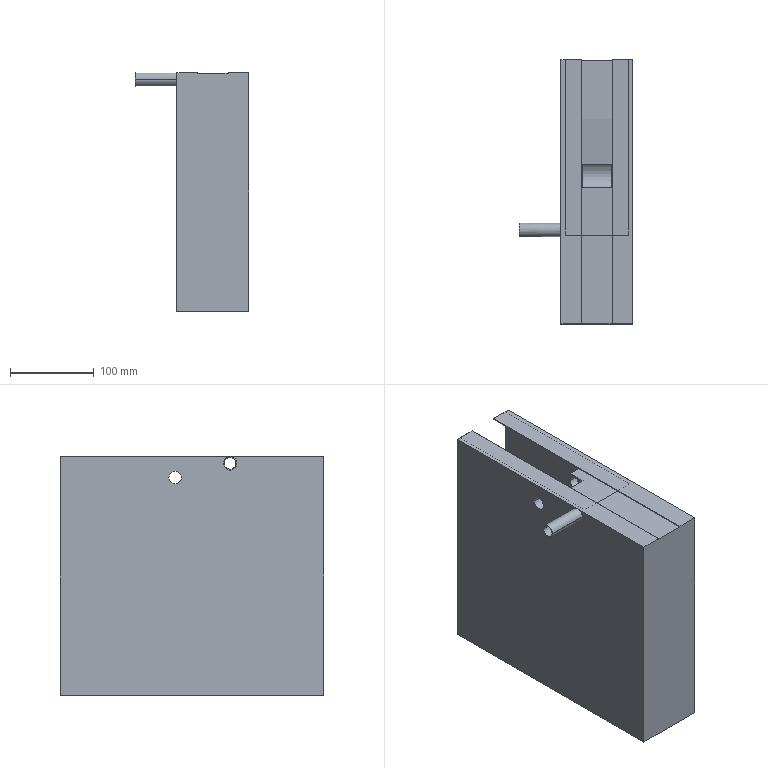Component | SolidWorks | HZ022-A001-E001-1 | 1 solid | 37 faces | box 136 x 315 x 285 mm | volume 5407462 mm3 | plane 25 | cylinder 12 | commonest cylinder face diameters 14 x4 15 x4 16 x2 35 x2 | material AL6061
build123d program:
from build123d import *
from build123d.topology import SkipClean

# Parameters (mm, degrees)
SKETCH1_6_W         = 285
SKETCH1_6_H         = 250
BOSS_EXTRUDE2_DEPTH = 5
BOSS_EXTRUDE3_DEPTH = 38
BOSS_EXTRUDE4_DEPTH = 20
SKETCH4_W           = 285
SKETCH4_H           = 250
BOSS_EXTRUDE5_DEPTH = 5
SKETCH5_R           = 17.5
CUT_EXTRUDE1_DEPTH  = 17.5
SKETCH6_R           = 7.5
CUT_EXTRUDE2_DEPTH  = 47.5
SKETCH7_R           = 7
CUT_EXTRUDE3_DEPTH  = 389.743
SKETCH8_R           = 8
SKETCH8_R_2         = 7
EXTRUDE_THIN1_DEPTH = 50
BOSS_EXTRUDE6_DEPTH = 65


with BuildPart() as part:
    # Sketch1_6 → Boss-Extrude2 (new body)
    with BuildSketch(Plane(origin=(0, 0, 0), x_dir=(1, 0, 0), z_dir=(0, 1, 0))):
        with Locations((142.5, 125)):
            Rectangle(SKETCH1_6_W, SKETCH1_6_H)
    extrude(amount=-BOSS_EXTRUDE2_DEPTH)

    # Sketch1_5 → Boss-Extrude3 (add)
    with BuildSketch(Plane(origin=(0, 0, 0), x_dir=(1, 0, 0), z_dir=(0, 1, 0))):
        Polygon((1, 40), (1, 0), (285, 0), (285, 250), (284, 250), (284, 179.778), (15, 120), (15, 40), align=None)
    boss_extrude3 = extrude(amount=BOSS_EXTRUDE3_DEPTH)

    # Sketch1_6 2 → Boss-Extrude4 (add)
    with BuildSketch(Plane(origin=(0, 0, 0), x_dir=(1, 0, 0), z_dir=(0, 1, 0))):
        Polygon((0, 250), (0, 0), (1, 0), (1, 40), (1, 250), align=None)
    boss_extrude4 = extrude(amount=BOSS_EXTRUDE4_DEPTH)

    # Mirror1: Boss-Extrude3, Boss-Extrude4 across plane
    add(boss_extrude3.mirror(Plane.ZX.offset(38)))
    add(boss_extrude4.mirror(Plane.ZX.offset(38)))

    # Sketch4 → Boss-Extrude5 (add)
    with BuildSketch(Plane(origin=(0, 76, 0), x_dir=(1, 0, 0), z_dir=(0, 1, 0))):
        with Locations((142.5, 125)):
            Rectangle(SKETCH4_W, SKETCH4_H)
    extrude(amount=BOSS_EXTRUDE5_DEPTH)

    # Sketch5 → Cut-Extrude1 (cut, symmetric)
    with BuildSketch(Plane(origin=(0, 38, 0), x_dir=(1, 0, 0), z_dir=(0, 1, 0))):
        with Locations((25, 112.5)):
            Circle(SKETCH5_R)
    extrude(amount=CUT_EXTRUDE1_DEPTH, both=True, mode=Mode.SUBTRACT)

    # Sketch6 → Cut-Extrude2 (cut, symmetric)
    with BuildSketch(Plane(origin=(0, 38, 0), x_dir=(1, 0, 0), z_dir=(0, 1, 0))):
        with Locations(Location((25, 112.5, 0), (0, 0, 270))):
            Circle(SKETCH6_R)
    extrude(amount=CUT_EXTRUDE2_DEPTH, both=True, mode=Mode.SUBTRACT)

    # Sketch7 → Cut-Extrude3 (cut, through all)
    with BuildSketch(Plane(origin=(0, 81, 0), x_dir=(1, 0, 0), z_dir=(0, 1, 0))):
        with Locations(Location((8, 47, 0), (0, 0, 270))):
            Circle(SKETCH7_R)
    extrude(amount=-CUT_EXTRUDE3_DEPTH, mode=Mode.SUBTRACT)

    # Sketch8 → Extrude-Thin1 (add)
    with SkipClean():  # the faces are left unmerged after this step: merging them gives an invalid solid
        with BuildSketch(Plane.XZ.offset(5)):
            with Locations((8, -47)):
                Circle(SKETCH8_R)
            with Locations((8, -47)):
                Circle(SKETCH8_R_2, mode=Mode.SUBTRACT)
        extrude(amount=EXTRUDE_THIN1_DEPTH)

    # Sketch9 → Boss-Extrude6 (add)
    with SkipClean():  # the faces are left unmerged after this step: merging them gives an invalid solid
        with BuildSketch(Plane.XY):
            Polygon((1, 20), (0, 20), (0, -5), (285, -5), (285, 81), (0, 81), (0, 56), (1, 56), align=None)
        extrude(amount=BOSS_EXTRUDE6_DEPTH)


solid = part.part

# Placed as in the assembly
solid = solid.moved(Location((-2.556, 79.652, 935), (90, 0, -90)))